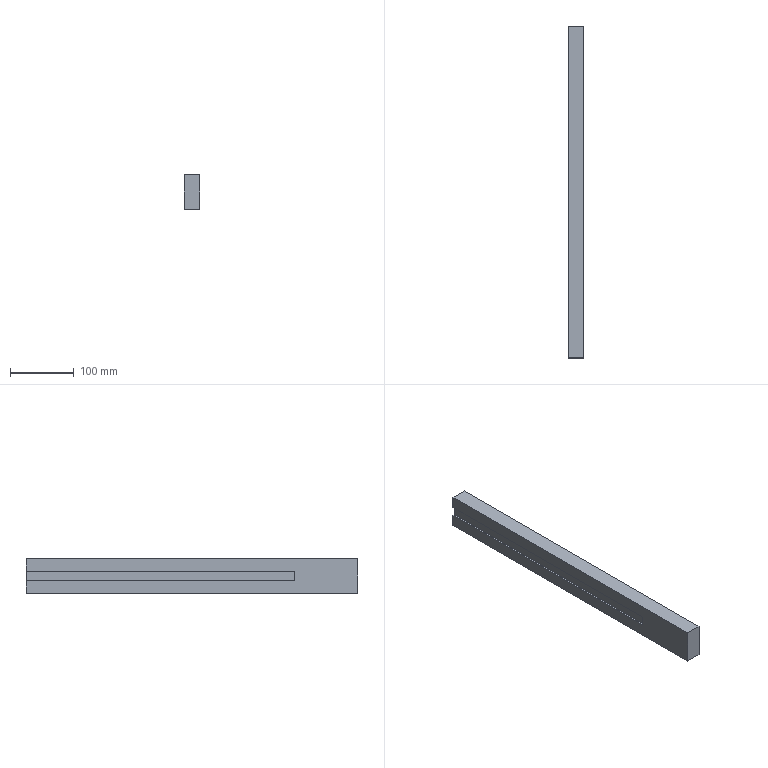Component | SolidWorks | FixedColumn-1 | 1 solid | 10 faces | box 25 x 520 x 54 mm | volume 683100 mm3 | plane 10
build123d program:
from build123d import *

# Parameters (mm, degrees)
SKETCH2_W           = 25
SKETCH2_H           = 54
BOSS_EXTRUDE1_DEPTH = 520
SKETCH3_W           = 420
SKETCH3_H           = 15
CUT_EXTRUDE1_DEPTH  = 3


with BuildPart() as part:
    # Sketch2 → Boss-Extrude1 (new body)
    with BuildSketch(Plane.XY):
        with Locations((96.375, -271.907)):
            Rectangle(SKETCH2_W, SKETCH2_H)
    extrude(amount=BOSS_EXTRUDE1_DEPTH)

    # Sketch3 → Cut-Extrude1 (cut)
    with BuildSketch(Plane.ZY.offset(-83.875)):
        with Locations((310, -271.907)):
            Rectangle(SKETCH3_W, SKETCH3_H)
    extrude(amount=-CUT_EXTRUDE1_DEPTH, mode=Mode.SUBTRACT)


solid = part.part

# Placed as in the assembly
solid = solid.moved(Location((-542.171, -147.651, -0.2817), (-90, 0, 0)))
STEP:
#1=COLOUR_RGB('',0.7922,0.8196,0.9333);
#2=FILL_AREA_STYLE_COLOUR('',#1);
#3=FILL_AREA_STYLE('',(#2));
#4=SURFACE_STYLE_FILL_AREA(#3);
#5=SURFACE_SIDE_STYLE('',(#4));
#6=SURFACE_STYLE_USAGE(.BOTH.,#5);
#7=PRESENTATION_STYLE_ASSIGNMENT((#6));
#8=CARTESIAN_POINT('',(-18.043,14.659,10.989));
#9=VERTEX_POINT('',#8);
#10=CARTESIAN_POINT('',(-18.043,14.659,11.757));
#11=VERTEX_POINT('',#10);
#12=CARTESIAN_POINT('',(-18.043,14.659,11.757));
#13=DIRECTION('',(-0.,0.,1.));
#14=VECTOR('',#13,39.37);
#15=LINE('',#12,#14);
#16=EDGE_CURVE('',#9,#11,#15,.T.);
#17=ORIENTED_EDGE('',*,*,#16,.F.);
#18=CARTESIAN_POINT('',(-18.043,-1.876,10.989));
#19=VERTEX_POINT('',#18);
#20=CARTESIAN_POINT('',(-18.043,14.659,10.989));
#21=DIRECTION('',(-0.,1.,-0.));
#22=VECTOR('',#21,39.37);
#23=LINE('',#20,#22);
#24=EDGE_CURVE('',#19,#9,#23,.T.);
#25=ORIENTED_EDGE('',*,*,#24,.F.);
#26=CARTESIAN_POINT('',(-18.043,-1.876,10.399));
#27=VERTEX_POINT('',#26);
#28=CARTESIAN_POINT('',(-18.043,-1.876,10.399));
#29=DIRECTION('',(-0.,0.,1.));
#30=VECTOR('',#29,39.37);
#31=LINE('',#28,#30);
#32=EDGE_CURVE('',#27,#19,#31,.T.);
#33=ORIENTED_EDGE('',*,*,#32,.F.);
#34=CARTESIAN_POINT('',(-18.043,14.659,10.399));
#35=VERTEX_POINT('',#34);
#36=CARTESIAN_POINT('',(-18.043,14.659,10.399));
#37=DIRECTION('',(0.,-1.,0.));
#38=VECTOR('',#37,39.37);
#39=LINE('',#36,#38);
#40=EDGE_CURVE('',#35,#27,#39,.T.);
#41=ORIENTED_EDGE('',*,*,#40,.F.);
#42=CARTESIAN_POINT('',(-18.043,14.659,9.631));
#43=VERTEX_POINT('',#42);
#44=CARTESIAN_POINT('',(-18.043,14.659,11.757));
#45=DIRECTION('',(-0.,0.,1.));
#46=VECTOR('',#45,39.37);
#47=LINE('',#44,#46);
#48=EDGE_CURVE('',#43,#35,#47,.T.);
#49=ORIENTED_EDGE('',*,*,#48,.F.);
#50=CARTESIAN_POINT('',(-18.043,-5.813,9.631));
#51=VERTEX_POINT('',#50);
#52=CARTESIAN_POINT('',(-18.043,14.659,9.631));
#53=DIRECTION('',(0.,-1.,0.));
#54=VECTOR('',#53,39.37);
#55=LINE('',#52,#54);
#56=EDGE_CURVE('',#43,#51,#55,.T.);
#57=ORIENTED_EDGE('',*,*,#56,.T.);
#58=CARTESIAN_POINT('',(-18.043,-5.813,11.757));
#59=VERTEX_POINT('',#58);
#60=CARTESIAN_POINT('',(-18.043,-5.813,11.757));
#61=DIRECTION('',(-0.,0.,1.));
#62=VECTOR('',#61,39.37);
#63=LINE('',#60,#62);
#64=EDGE_CURVE('',#51,#59,#63,.T.);
#65=ORIENTED_EDGE('',*,*,#64,.T.);
#66=CARTESIAN_POINT('',(-18.043,14.659,11.757));
#67=DIRECTION('',(0.,-1.,0.));
#68=VECTOR('',#67,39.37);
#69=LINE('',#66,#68);
#70=EDGE_CURVE('',#11,#59,#69,.T.);
#71=ORIENTED_EDGE('',*,*,#70,.F.);
#72=EDGE_LOOP('',(#17,#25,#33,#41,#49,#57,#65,#71));
#73=FACE_OUTER_BOUND('',#72,.T.);
#74=CARTESIAN_POINT('',(-18.043,14.659,11.757));
#75=DIRECTION('',(1.,0.,0.));
#76=DIRECTION('',(0.,-1.,0.));
#77=AXIS2_PLACEMENT_3D('',#74,#75,#76);
#78=PLANE('',#77);
#79=ADVANCED_FACE('',(#73),#78,.F.);
#80=CARTESIAN_POINT('',(-17.059,-5.813,11.757));
#81=VERTEX_POINT('',#80);
#82=CARTESIAN_POINT('',(-18.043,-5.813,11.757));
#83=DIRECTION('',(1.,0.,0.));
#84=VECTOR('',#83,39.37);
#85=LINE('',#82,#84);
#86=EDGE_CURVE('',#59,#81,#85,.T.);
#87=ORIENTED_EDGE('',*,*,#86,.T.);
#88=CARTESIAN_POINT('',(-17.059,14.659,11.757));
#89=VERTEX_POINT('',#88);
#90=CARTESIAN_POINT('',(-17.059,14.659,11.757));
#91=DIRECTION('',(0.,-1.,0.));
#92=VECTOR('',#91,39.37);
#93=LINE('',#90,#92);
#94=EDGE_CURVE('',#89,#81,#93,.T.);
#95=ORIENTED_EDGE('',*,*,#94,.F.);
#96=CARTESIAN_POINT('',(-18.043,14.659,11.757));
#97=DIRECTION('',(1.,0.,0.));
#98=VECTOR('',#97,39.37);
#99=LINE('',#96,#98);
#100=EDGE_CURVE('',#11,#89,#99,.T.);
#101=ORIENTED_EDGE('',*,*,#100,.F.);
#102=ORIENTED_EDGE('',*,*,#70,.T.);
#103=EDGE_LOOP('',(#87,#95,#101,#102));
#104=FACE_OUTER_BOUND('',#103,.T.);
#105=CARTESIAN_POINT('',(-18.043,14.659,11.757));
#106=DIRECTION('',(0.,-0.,-1.));
#107=DIRECTION('',(-0.,1.,-0.));
#108=AXIS2_PLACEMENT_3D('',#105,#106,#107);
#109=PLANE('',#108);
#110=ADVANCED_FACE('',(#104),#109,.F.);
#111=CARTESIAN_POINT('',(-17.059,-5.813,9.631));
#112=VERTEX_POINT('',#111);
#113=CARTESIAN_POINT('',(-17.059,-5.813,11.757));
#114=DIRECTION('',(0.,-0.,-1.));
#115=VECTOR('',#114,39.37);
#116=LINE('',#113,#115);
#117=EDGE_CURVE('',#81,#112,#116,.T.);
#118=ORIENTED_EDGE('',*,*,#117,.T.);
#119=CARTESIAN_POINT('',(-17.059,14.659,9.631));
#120=VERTEX_POINT('',#119);
#121=CARTESIAN_POINT('',(-17.059,14.659,9.631));
#122=DIRECTION('',(0.,-1.,0.));
#123=VECTOR('',#122,39.37);
#124=LINE('',#121,#123);
#125=EDGE_CURVE('',#120,#112,#124,.T.);
#126=ORIENTED_EDGE('',*,*,#125,.F.);
#127=CARTESIAN_POINT('',(-17.059,14.659,11.757));
#128=DIRECTION('',(0.,-0.,-1.));
#129=VECTOR('',#128,39.37);
#130=LINE('',#127,#129);
#131=EDGE_CURVE('',#89,#120,#130,.T.);
#132=ORIENTED_EDGE('',*,*,#131,.F.);
#133=ORIENTED_EDGE('',*,*,#94,.T.);
#134=EDGE_LOOP('',(#118,#126,#132,#133));
#135=FACE_OUTER_BOUND('',#134,.T.);
#136=CARTESIAN_POINT('',(-17.059,14.659,11.757));
#137=DIRECTION('',(-1.,-0.,-0.));
#138=DIRECTION('',(-0.,1.,-0.));
#139=AXIS2_PLACEMENT_3D('',#136,#137,#138);
#140=PLANE('',#139);
#141=ADVANCED_FACE('',(#135),#140,.F.);
#142=CARTESIAN_POINT('',(-18.043,-5.813,9.631));
#143=DIRECTION('',(-1.,-0.,-0.));
#144=VECTOR('',#143,39.37);
#145=LINE('',#142,#144);
#146=EDGE_CURVE('',#112,#51,#145,.T.);
#147=ORIENTED_EDGE('',*,*,#146,.T.);
#148=ORIENTED_EDGE('',*,*,#56,.F.);
#149=CARTESIAN_POINT('',(-18.043,14.659,9.631));
#150=DIRECTION('',(-1.,-0.,-0.));
#151=VECTOR('',#150,39.37);
#152=LINE('',#149,#151);
#153=EDGE_CURVE('',#120,#43,#152,.T.);
#154=ORIENTED_EDGE('',*,*,#153,.F.);
#155=ORIENTED_EDGE('',*,*,#125,.T.);
#156=EDGE_LOOP('',(#147,#148,#154,#155));
#157=FACE_OUTER_BOUND('',#156,.T.);
#158=CARTESIAN_POINT('',(-18.043,14.659,9.631));
#159=DIRECTION('',(-0.,0.,1.));
#160=DIRECTION('',(0.,-1.,0.));
#161=AXIS2_PLACEMENT_3D('',#158,#159,#160);
#162=PLANE('',#161);
#163=ADVANCED_FACE('',(#157),#162,.F.);
#164=CARTESIAN_POINT('',(-17.925,14.659,10.989));
#165=VERTEX_POINT('',#164);
#166=CARTESIAN_POINT('',(-17.925,14.659,10.399));
#167=VERTEX_POINT('',#166);
#168=CARTESIAN_POINT('',(-17.925,14.659,10.399));
#169=DIRECTION('',(0.,-0.,-1.));
#170=VECTOR('',#169,39.37);
#171=LINE('',#168,#170);
#172=EDGE_CURVE('',#165,#167,#171,.T.);
#173=ORIENTED_EDGE('',*,*,#172,.F.);
#174=CARTESIAN_POINT('',(-17.925,14.659,10.989));
#175=DIRECTION('',(-1.,-0.,-0.));
#176=VECTOR('',#175,39.37);
#177=LINE('',#174,#176);
#178=EDGE_CURVE('',#165,#9,#177,.T.);
#179=ORIENTED_EDGE('',*,*,#178,.T.);
#180=ORIENTED_EDGE('',*,*,#16,.T.);
#181=ORIENTED_EDGE('',*,*,#100,.T.);
#182=ORIENTED_EDGE('',*,*,#131,.T.);
#183=ORIENTED_EDGE('',*,*,#153,.T.);
#184=ORIENTED_EDGE('',*,*,#48,.T.);
#185=CARTESIAN_POINT('',(-17.925,14.659,10.399));
#186=DIRECTION('',(-1.,-0.,-0.));
#187=VECTOR('',#186,39.37);
#188=LINE('',#185,#187);
#189=EDGE_CURVE('',#167,#35,#188,.T.);
#190=ORIENTED_EDGE('',*,*,#189,.F.);
#191=EDGE_LOOP('',(#173,#179,#180,#181,#182,#183,#184,#190));
#192=FACE_OUTER_BOUND('',#191,.T.);
#193=CARTESIAN_POINT('',(-21.345,14.659,-0.01109));
#194=DIRECTION('',(0.,-1.,0.));
#195=DIRECTION('',(-1.,-0.,-0.));
#196=AXIS2_PLACEMENT_3D('',#193,#194,#195);
#197=PLANE('',#196);
#198=ADVANCED_FACE('',(#192),#197,.F.);
#199=ORIENTED_EDGE('',*,*,#64,.F.);
#200=ORIENTED_EDGE('',*,*,#146,.F.);
#201=ORIENTED_EDGE('',*,*,#117,.F.);
#202=ORIENTED_EDGE('',*,*,#86,.F.);
#203=EDGE_LOOP('',(#199,#200,#201,#202));
#204=FACE_OUTER_BOUND('',#203,.T.);
#205=CARTESIAN_POINT('',(-21.345,-5.813,-0.01109));
#206=DIRECTION('',(0.,-1.,0.));
#207=DIRECTION('',(-1.,-0.,-0.));
#208=AXIS2_PLACEMENT_3D('',#205,#206,#207);
#209=PLANE('',#208);
#210=ADVANCED_FACE('',(#204),#209,.T.);
#211=ORIENTED_EDGE('',*,*,#24,.T.);
#212=ORIENTED_EDGE('',*,*,#178,.F.);
#213=CARTESIAN_POINT('',(-17.925,-1.876,10.989));
#214=VERTEX_POINT('',#213);
#215=CARTESIAN_POINT('',(-17.925,14.659,10.989));
#216=DIRECTION('',(-0.,1.,-0.));
#217=VECTOR('',#216,39.37);
#218=LINE('',#215,#217);
#219=EDGE_CURVE('',#214,#165,#218,.T.);
#220=ORIENTED_EDGE('',*,*,#219,.F.);
#221=CARTESIAN_POINT('',(-17.925,-1.876,10.989));
#222=DIRECTION('',(-1.,-0.,-0.));
#223=VECTOR('',#222,39.37);
#224=LINE('',#221,#223);
#225=EDGE_CURVE('',#214,#19,#224,.T.);
#226=ORIENTED_EDGE('',*,*,#225,.T.);
#227=EDGE_LOOP('',(#211,#212,#220,#226));
#228=FACE_OUTER_BOUND('',#227,.T.);
#229=CARTESIAN_POINT('',(-17.925,14.659,10.989));
#230=DIRECTION('',(-0.,0.,1.));
#231=DIRECTION('',(0.,-1.,0.));
#232=AXIS2_PLACEMENT_3D('',#229,#230,#231);
#233=PLANE('',#232);
#234=ADVANCED_FACE('',(#228),#233,.F.);
#235=ORIENTED_EDGE('',*,*,#32,.T.);
#236=ORIENTED_EDGE('',*,*,#225,.F.);
#237=CARTESIAN_POINT('',(-17.925,-1.876,10.399));
#238=VERTEX_POINT('',#237);
#239=CARTESIAN_POINT('',(-17.925,-1.876,10.399));
#240=DIRECTION('',(-0.,0.,1.));
#241=VECTOR('',#240,39.37);
#242=LINE('',#239,#241);
#243=EDGE_CURVE('',#238,#214,#242,.T.);
#244=ORIENTED_EDGE('',*,*,#243,.F.);
#245=CARTESIAN_POINT('',(-17.925,-1.876,10.399));
#246=DIRECTION('',(-1.,-0.,-0.));
#247=VECTOR('',#246,39.37);
#248=LINE('',#245,#247);
#249=EDGE_CURVE('',#238,#27,#248,.T.);
#250=ORIENTED_EDGE('',*,*,#249,.T.);
#251=EDGE_LOOP('',(#235,#236,#244,#250));
#252=FACE_OUTER_BOUND('',#251,.T.);
#253=CARTESIAN_POINT('',(-17.925,-1.876,10.399));
#254=DIRECTION('',(0.,-1.,0.));
#255=DIRECTION('',(-1.,-0.,-0.));
#256=AXIS2_PLACEMENT_3D('',#253,#254,#255);
#257=PLANE('',#256);
#258=ADVANCED_FACE('',(#252),#257,.F.);
#259=ORIENTED_EDGE('',*,*,#40,.T.);
#260=ORIENTED_EDGE('',*,*,#249,.F.);
#261=CARTESIAN_POINT('',(-17.925,14.659,10.399));
#262=DIRECTION('',(0.,-1.,0.));
#263=VECTOR('',#262,39.37);
#264=LINE('',#261,#263);
#265=EDGE_CURVE('',#167,#238,#264,.T.);
#266=ORIENTED_EDGE('',*,*,#265,.F.);
#267=ORIENTED_EDGE('',*,*,#189,.T.);
#268=EDGE_LOOP('',(#259,#260,#266,#267));
#269=FACE_OUTER_BOUND('',#268,.T.);
#270=CARTESIAN_POINT('',(-17.925,14.659,10.399));
#271=DIRECTION('',(0.,-0.,-1.));
#272=DIRECTION('',(-0.,1.,-0.));
#273=AXIS2_PLACEMENT_3D('',#270,#271,#272);
#274=PLANE('',#273);
#275=ADVANCED_FACE('',(#269),#274,.F.);
#276=ORIENTED_EDGE('',*,*,#172,.T.);
#277=ORIENTED_EDGE('',*,*,#265,.T.);
#278=ORIENTED_EDGE('',*,*,#243,.T.);
#279=ORIENTED_EDGE('',*,*,#219,.T.);
#280=EDGE_LOOP('',(#276,#277,#278,#279));
#281=FACE_OUTER_BOUND('',#280,.T.);
#282=CARTESIAN_POINT('',(-17.925,-5.813,-0.01109));
#283=DIRECTION('',(1.,0.,0.));
#284=DIRECTION('',(0.,-1.,0.));
#285=AXIS2_PLACEMENT_3D('',#282,#283,#284);
#286=PLANE('',#285);
#287=ADVANCED_FACE('',(#281),#286,.F.);
#288=CLOSED_SHELL('',(#79,#110,#141,#163,#198,#210,#234,#258,#275,#287));
#289=MANIFOLD_SOLID_BREP('',#288);
#290=STYLED_ITEM('',(#7),#289);
#291=PRESENTATION_LAYER_ASSIGNMENT('','',(#290));
#292=(LENGTH_UNIT()NAMED_UNIT(*)SI_UNIT($,.METRE.));
#293=LENGTH_MEASURE_WITH_UNIT(LENGTH_MEASURE(0.0254),#292);
#294=DIMENSIONAL_EXPONENTS(1.,0.,0.,0.,0.,0.,0.);
#295=(CONVERSION_BASED_UNIT('',#293)LENGTH_UNIT()NAMED_UNIT(#294));
#296=UNCERTAINTY_MEASURE_WITH_UNIT(LENGTH_MEASURE(0.00001),#295,'','');
#297=(NAMED_UNIT(*)PLANE_ANGLE_UNIT()SI_UNIT($,.RADIAN.));
#298=(NAMED_UNIT(*)SI_UNIT($,.STERADIAN.)SOLID_ANGLE_UNIT());
#299=(GEOMETRIC_REPRESENTATION_CONTEXT(3)GLOBAL_UNCERTAINTY_ASSIGNED_CONTEXT((#296))GLOBAL_UNIT_ASSIGNED_CONTEXT((#295,#297,#298))REPRESENTATION_CONTEXT('',''));
#300=MECHANICAL_DESIGN_GEOMETRIC_PRESENTATION_REPRESENTATION('',(#290),#299);
#301=CARTESIAN_POINT('',(0.,0.,0.));
#302=DIRECTION('',(0.,0.,1.));
#303=DIRECTION('',(1.,0.,0.));
#304=AXIS2_PLACEMENT_3D('',#301,#302,#303);
#305=(LENGTH_UNIT()NAMED_UNIT(*)SI_UNIT($,.METRE.));
#306=LENGTH_MEASURE_WITH_UNIT(LENGTH_MEASURE(0.0254),#305);
#307=DIMENSIONAL_EXPONENTS(1.,0.,0.,0.,0.,0.,0.);
#308=(CONVERSION_BASED_UNIT('',#306)LENGTH_UNIT()NAMED_UNIT(#307));
#309=UNCERTAINTY_MEASURE_WITH_UNIT(LENGTH_MEASURE(0.00001),#308,'','');
#310=(NAMED_UNIT(*)PLANE_ANGLE_UNIT()SI_UNIT($,.RADIAN.));
#311=(NAMED_UNIT(*)SI_UNIT($,.STERADIAN.)SOLID_ANGLE_UNIT());
#312=(GEOMETRIC_REPRESENTATION_CONTEXT(3)GLOBAL_UNCERTAINTY_ASSIGNED_CONTEXT((#309))GLOBAL_UNIT_ASSIGNED_CONTEXT((#308,#310,#311))REPRESENTATION_CONTEXT('',''));
#313=ADVANCED_BREP_SHAPE_REPRESENTATION('',(#289,#304),#312);